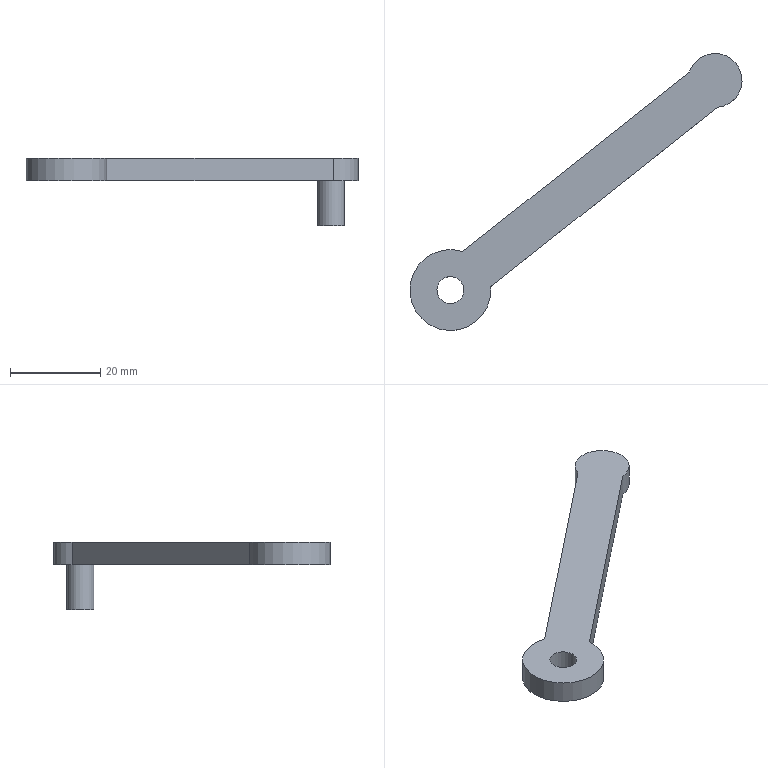Component | NX | CONN_ARM | 1 solid | 9 faces | box 73.78 x 61.58 x 15 mm | volume 5043 mm3 | plane 5 | cylinder 4 | commonest cylinder face diameters 6 x2 12 x1 18 x1
STEP:
#1=CARTESIAN_POINT('',(0.,0.,0.));
#2=DIRECTION('',(0.,0.,1.));
#3=DIRECTION('',(1.,0.,0.));
#4=AXIS2_PLACEMENT_3D('',#1,#2,#3);
#5=CARTESIAN_POINT('',(-109.814,-45.848,12.5));
#6=VERTEX_POINT('',#5);
#7=CARTESIAN_POINT('',(-59.494,-5.979,12.5));
#8=VERTEX_POINT('',#7);
#9=CARTESIAN_POINT('',(-109.814,-45.848,12.5));
#10=DIRECTION('',(0.7838,0.621,0.));
#11=VECTOR('',#10,1.);
#12=LINE('',#9,#11);
#13=CARTESIAN_POINT('',(-109.814,-45.848,7.5));
#14=DIRECTION('',(0.621,-0.7838,0.));
#15=DIRECTION('',(0.,0.,-1.));
#16=AXIS2_PLACEMENT_3D('',#13,#14,#15);
#17=PLANE('',#16);
#18=CARTESIAN_POINT('',(-5.,0.));
#19=DIRECTION('',(0.,1.));
#20=VECTOR('',#19,1.);
#21=LINE('',#18,#20);
#22=(GEOMETRIC_REPRESENTATION_CONTEXT(2)PARAMETRIC_REPRESENTATION_CONTEXT()REPRESENTATION_CONTEXT('',''));
#23=DEFINITIONAL_REPRESENTATION('',(#21),#22);
#24=PCURVE('',#17,#23);
#25=CARTESIAN_POINT('',(-60.,-0.,12.5));
#26=DIRECTION('',(0.,0.,1.));
#27=DIRECTION('',(-0.7838,-0.621,0.));
#28=AXIS2_PLACEMENT_3D('',#25,#26,#27);
#29=PLANE('',#28);
#30=CARTESIAN_POINT('',(67.517,5.));
#31=DIRECTION('',(-1.,0.));
#32=VECTOR('',#31,1.);
#33=LINE('',#30,#32);
#34=(GEOMETRIC_REPRESENTATION_CONTEXT(2)PARAMETRIC_REPRESENTATION_CONTEXT()REPRESENTATION_CONTEXT('',''));
#35=DEFINITIONAL_REPRESENTATION('',(#33),#34);
#36=PCURVE('',#29,#35);
#37=SURFACE_CURVE('',#12,(#24,#36),.PCURVE_S1.);
#38=EDGE_CURVE('',#6,#8,#37,.T.);
#39=ORIENTED_EDGE('',*,*,#38,.F.);
#40=CARTESIAN_POINT('',(-109.814,-45.848,7.5));
#41=VERTEX_POINT('',#40);
#42=CARTESIAN_POINT('',(-109.814,-45.848,7.5));
#43=DIRECTION('',(0.,0.,1.));
#44=VECTOR('',#43,1.);
#45=LINE('',#42,#44);
#46=CARTESIAN_POINT('',(0.,0.));
#47=DIRECTION('',(-1.,0.));
#48=VECTOR('',#47,1.);
#49=LINE('',#46,#48);
#50=(GEOMETRIC_REPRESENTATION_CONTEXT(2)PARAMETRIC_REPRESENTATION_CONTEXT()REPRESENTATION_CONTEXT('',''));
#51=DEFINITIONAL_REPRESENTATION('',(#49),#50);
#52=PCURVE('',#17,#51);
#53=CARTESIAN_POINT('',(-118.784,-46.577,7.5));
#54=DIRECTION('',(0.,0.,1.));
#55=DIRECTION('',(-0.7838,-0.621,0.));
#56=AXIS2_PLACEMENT_3D('',#53,#54,#55);
#57=CYLINDRICAL_SURFACE('',#56,9.);
#58=CARTESIAN_POINT('',(8.836,0.));
#59=DIRECTION('',(0.,1.));
#60=VECTOR('',#59,1.);
#61=LINE('',#58,#60);
#62=(GEOMETRIC_REPRESENTATION_CONTEXT(2)PARAMETRIC_REPRESENTATION_CONTEXT()REPRESENTATION_CONTEXT('',''));
#63=DEFINITIONAL_REPRESENTATION('',(#61),#62);
#64=PCURVE('',#57,#63);
#65=SURFACE_CURVE('',#45,(#52,#64),.PCURVE_S1.);
#66=EDGE_CURVE('',#41,#6,#65,.T.);
#67=ORIENTED_EDGE('',*,*,#66,.F.);
#68=CARTESIAN_POINT('',(-59.494,-5.979,7.5));
#69=VERTEX_POINT('',#68);
#70=CARTESIAN_POINT('',(-109.814,-45.848,7.5));
#71=DIRECTION('',(0.7838,0.621,0.));
#72=VECTOR('',#71,1.);
#73=LINE('',#70,#72);
#74=CARTESIAN_POINT('',(0.,0.));
#75=DIRECTION('',(0.,1.));
#76=VECTOR('',#75,1.);
#77=LINE('',#74,#76);
#78=(GEOMETRIC_REPRESENTATION_CONTEXT(2)PARAMETRIC_REPRESENTATION_CONTEXT()REPRESENTATION_CONTEXT('',''));
#79=DEFINITIONAL_REPRESENTATION('',(#77),#78);
#80=PCURVE('',#17,#79);
#81=CARTESIAN_POINT('',(-60.,-0.,7.5));
#82=DIRECTION('',(0.,0.,1.));
#83=DIRECTION('',(-0.7838,-0.621,0.));
#84=AXIS2_PLACEMENT_3D('',#81,#82,#83);
#85=PLANE('',#84);
#86=CARTESIAN_POINT('',(67.517,5.));
#87=DIRECTION('',(-1.,0.));
#88=VECTOR('',#87,1.);
#89=LINE('',#86,#88);
#90=(GEOMETRIC_REPRESENTATION_CONTEXT(2)PARAMETRIC_REPRESENTATION_CONTEXT()REPRESENTATION_CONTEXT('',''));
#91=DEFINITIONAL_REPRESENTATION('',(#89),#90);
#92=PCURVE('',#85,#91);
#93=SURFACE_CURVE('',#73,(#80,#92),.PCURVE_S1.);
#94=EDGE_CURVE('',#41,#69,#93,.T.);
#95=ORIENTED_EDGE('',*,*,#94,.T.);
#96=CARTESIAN_POINT('',(-59.494,-5.979,7.5));
#97=DIRECTION('',(0.,0.,1.));
#98=VECTOR('',#97,1.);
#99=LINE('',#96,#98);
#100=CARTESIAN_POINT('',(0.,64.2));
#101=DIRECTION('',(-1.,0.));
#102=VECTOR('',#101,1.);
#103=LINE('',#100,#102);
#104=(GEOMETRIC_REPRESENTATION_CONTEXT(2)PARAMETRIC_REPRESENTATION_CONTEXT()REPRESENTATION_CONTEXT('',''));
#105=DEFINITIONAL_REPRESENTATION('',(#103),#104);
#106=PCURVE('',#17,#105);
#107=CARTESIAN_POINT('',(-60.,-0.,7.5));
#108=DIRECTION('',(0.,0.,1.));
#109=DIRECTION('',(-0.7838,-0.621,0.));
#110=AXIS2_PLACEMENT_3D('',#107,#108,#109);
#111=CYLINDRICAL_SURFACE('',#110,6.);
#112=CARTESIAN_POINT('',(0.9851,0.));
#113=DIRECTION('',(0.,1.));
#114=VECTOR('',#113,1.);
#115=LINE('',#112,#114);
#116=(GEOMETRIC_REPRESENTATION_CONTEXT(2)PARAMETRIC_REPRESENTATION_CONTEXT()REPRESENTATION_CONTEXT('',''));
#117=DEFINITIONAL_REPRESENTATION('',(#115),#116);
#118=PCURVE('',#111,#117);
#119=SURFACE_CURVE('',#99,(#106,#118),.PCURVE_S1.);
#120=EDGE_CURVE('',#69,#8,#119,.T.);
#121=ORIENTED_EDGE('',*,*,#120,.T.);
#122=EDGE_LOOP('',(#39,#67,#95,#121));
#123=FACE_BOUND('',#122,.T.);
#124=ADVANCED_FACE('',(#123),#17,.T.);
#125=CARTESIAN_POINT('',(-65.705,1.859,12.5));
#126=VERTEX_POINT('',#125);
#127=CARTESIAN_POINT('',(-60.,-0.,12.5));
#128=DIRECTION('',(0.,0.,1.));
#129=DIRECTION('',(0.7838,0.621,0.));
#130=AXIS2_PLACEMENT_3D('',#127,#128,#129);
#131=CIRCLE('',#130,6.);
#132=CARTESIAN_POINT('',(-3.142,5.));
#133=DIRECTION('',(1.,0.));
#134=VECTOR('',#133,1.);
#135=LINE('',#132,#134);
#136=(GEOMETRIC_REPRESENTATION_CONTEXT(2)PARAMETRIC_REPRESENTATION_CONTEXT()REPRESENTATION_CONTEXT('',''));
#137=DEFINITIONAL_REPRESENTATION('',(#135),#136);
#138=PCURVE('',#111,#137);
#139=CARTESIAN_POINT('',(0.,0.));
#140=DIRECTION('',(-1.,0.));
#141=AXIS2_PLACEMENT_2D('',#139,#140);
#142=CIRCLE('',#141,6.);
#143=(GEOMETRIC_REPRESENTATION_CONTEXT(2)PARAMETRIC_REPRESENTATION_CONTEXT()REPRESENTATION_CONTEXT('',''));
#144=DEFINITIONAL_REPRESENTATION('',(#142),#143);
#145=PCURVE('',#29,#144);
#146=SURFACE_CURVE('',#131,(#138,#145),.PCURVE_S1.);
#147=EDGE_CURVE('',#8,#126,#146,.T.);
#148=ORIENTED_EDGE('',*,*,#147,.F.);
#149=ORIENTED_EDGE('',*,*,#120,.F.);
#150=CARTESIAN_POINT('',(-65.705,1.859,7.5));
#151=VERTEX_POINT('',#150);
#152=CARTESIAN_POINT('',(-60.,-0.,7.5));
#153=DIRECTION('',(0.,0.,1.));
#154=DIRECTION('',(0.7838,0.621,0.));
#155=AXIS2_PLACEMENT_3D('',#152,#153,#154);
#156=CIRCLE('',#155,6.);
#157=CARTESIAN_POINT('',(-3.142,0.));
#158=DIRECTION('',(1.,0.));
#159=VECTOR('',#158,1.);
#160=LINE('',#157,#159);
#161=(GEOMETRIC_REPRESENTATION_CONTEXT(2)PARAMETRIC_REPRESENTATION_CONTEXT()REPRESENTATION_CONTEXT('',''));
#162=DEFINITIONAL_REPRESENTATION('',(#160),#161);
#163=PCURVE('',#111,#162);
#164=CARTESIAN_POINT('',(0.,0.));
#165=DIRECTION('',(-1.,0.));
#166=AXIS2_PLACEMENT_2D('',#164,#165);
#167=CIRCLE('',#166,6.);
#168=(GEOMETRIC_REPRESENTATION_CONTEXT(2)PARAMETRIC_REPRESENTATION_CONTEXT()REPRESENTATION_CONTEXT('',''));
#169=DEFINITIONAL_REPRESENTATION('',(#167),#168);
#170=PCURVE('',#85,#169);
#171=SURFACE_CURVE('',#156,(#163,#170),.PCURVE_S1.);
#172=EDGE_CURVE('',#69,#151,#171,.T.);
#173=ORIENTED_EDGE('',*,*,#172,.T.);
#174=CARTESIAN_POINT('',(-65.705,1.859,7.5));
#175=DIRECTION('',(0.,0.,1.));
#176=VECTOR('',#175,1.);
#177=LINE('',#174,#176);
#178=CARTESIAN_POINT('',(5.298,0.));
#179=DIRECTION('',(0.,1.));
#180=VECTOR('',#179,1.);
#181=LINE('',#178,#180);
#182=(GEOMETRIC_REPRESENTATION_CONTEXT(2)PARAMETRIC_REPRESENTATION_CONTEXT()REPRESENTATION_CONTEXT('',''));
#183=DEFINITIONAL_REPRESENTATION('',(#181),#182);
#184=PCURVE('',#111,#183);
#185=CARTESIAN_POINT('',(-65.705,1.859,7.5));
#186=DIRECTION('',(-0.621,0.7838,0.));
#187=DIRECTION('',(0.,0.,1.));
#188=AXIS2_PLACEMENT_3D('',#185,#186,#187);
#189=PLANE('',#188);
#190=CARTESIAN_POINT('',(0.,0.));
#191=DIRECTION('',(1.,0.));
#192=VECTOR('',#191,1.);
#193=LINE('',#190,#192);
#194=(GEOMETRIC_REPRESENTATION_CONTEXT(2)PARAMETRIC_REPRESENTATION_CONTEXT()REPRESENTATION_CONTEXT('',''));
#195=DEFINITIONAL_REPRESENTATION('',(#193),#194);
#196=PCURVE('',#189,#195);
#197=SURFACE_CURVE('',#177,(#184,#196),.PCURVE_S1.);
#198=EDGE_CURVE('',#151,#126,#197,.T.);
#199=ORIENTED_EDGE('',*,*,#198,.T.);
#200=EDGE_LOOP('',(#148,#149,#173,#199));
#201=FACE_BOUND('',#200,.T.);
#202=ADVANCED_FACE('',(#201),#111,.T.);
#203=CARTESIAN_POINT('',(-116.024,-38.011,12.5));
#204=VERTEX_POINT('',#203);
#205=CARTESIAN_POINT('',(-65.705,1.859,12.5));
#206=DIRECTION('',(-0.7838,-0.621,0.));
#207=VECTOR('',#206,1.);
#208=LINE('',#205,#207);
#209=CARTESIAN_POINT('',(5.,0.));
#210=DIRECTION('',(0.,-1.));
#211=VECTOR('',#210,1.);
#212=LINE('',#209,#211);
#213=(GEOMETRIC_REPRESENTATION_CONTEXT(2)PARAMETRIC_REPRESENTATION_CONTEXT()REPRESENTATION_CONTEXT('',''));
#214=DEFINITIONAL_REPRESENTATION('',(#212),#213);
#215=PCURVE('',#189,#214);
#216=CARTESIAN_POINT('',(3.317,-5.));
#217=DIRECTION('',(1.,0.));
#218=VECTOR('',#217,1.);
#219=LINE('',#216,#218);
#220=(GEOMETRIC_REPRESENTATION_CONTEXT(2)PARAMETRIC_REPRESENTATION_CONTEXT()REPRESENTATION_CONTEXT('',''));
#221=DEFINITIONAL_REPRESENTATION('',(#219),#220);
#222=PCURVE('',#29,#221);
#223=SURFACE_CURVE('',#208,(#215,#222),.PCURVE_S1.);
#224=EDGE_CURVE('',#126,#204,#223,.T.);
#225=ORIENTED_EDGE('',*,*,#224,.F.);
#226=ORIENTED_EDGE('',*,*,#198,.F.);
#227=CARTESIAN_POINT('',(-116.024,-38.011,7.5));
#228=VERTEX_POINT('',#227);
#229=CARTESIAN_POINT('',(-65.705,1.859,7.5));
#230=DIRECTION('',(-0.7838,-0.621,0.));
#231=VECTOR('',#230,1.);
#232=LINE('',#229,#231);
#233=CARTESIAN_POINT('',(0.,0.));
#234=DIRECTION('',(0.,-1.));
#235=VECTOR('',#234,1.);
#236=LINE('',#233,#235);
#237=(GEOMETRIC_REPRESENTATION_CONTEXT(2)PARAMETRIC_REPRESENTATION_CONTEXT()REPRESENTATION_CONTEXT('',''));
#238=DEFINITIONAL_REPRESENTATION('',(#236),#237);
#239=PCURVE('',#189,#238);
#240=CARTESIAN_POINT('',(3.317,-5.));
#241=DIRECTION('',(1.,0.));
#242=VECTOR('',#241,1.);
#243=LINE('',#240,#242);
#244=(GEOMETRIC_REPRESENTATION_CONTEXT(2)PARAMETRIC_REPRESENTATION_CONTEXT()REPRESENTATION_CONTEXT('',''));
#245=DEFINITIONAL_REPRESENTATION('',(#243),#244);
#246=PCURVE('',#85,#245);
#247=SURFACE_CURVE('',#232,(#239,#246),.PCURVE_S1.);
#248=EDGE_CURVE('',#151,#228,#247,.T.);
#249=ORIENTED_EDGE('',*,*,#248,.T.);
#250=CARTESIAN_POINT('',(-116.024,-38.011,7.5));
#251=DIRECTION('',(0.,0.,1.));
#252=VECTOR('',#251,1.);
#253=LINE('',#250,#252);
#254=CARTESIAN_POINT('',(0.,-64.2));
#255=DIRECTION('',(1.,0.));
#256=VECTOR('',#255,1.);
#257=LINE('',#254,#256);
#258=(GEOMETRIC_REPRESENTATION_CONTEXT(2)PARAMETRIC_REPRESENTATION_CONTEXT()REPRESENTATION_CONTEXT('',''));
#259=DEFINITIONAL_REPRESENTATION('',(#257),#258);
#260=PCURVE('',#189,#259);
#261=CARTESIAN_POINT('',(3.731,0.));
#262=DIRECTION('',(0.,1.));
#263=VECTOR('',#262,1.);
#264=LINE('',#261,#263);
#265=(GEOMETRIC_REPRESENTATION_CONTEXT(2)PARAMETRIC_REPRESENTATION_CONTEXT()REPRESENTATION_CONTEXT('',''));
#266=DEFINITIONAL_REPRESENTATION('',(#264),#265);
#267=PCURVE('',#57,#266);
#268=SURFACE_CURVE('',#253,(#260,#267),.PCURVE_S1.);
#269=EDGE_CURVE('',#228,#204,#268,.T.);
#270=ORIENTED_EDGE('',*,*,#269,.T.);
#271=EDGE_LOOP('',(#225,#226,#249,#270));
#272=FACE_BOUND('',#271,.T.);
#273=ADVANCED_FACE('',(#272),#189,.T.);
#274=CARTESIAN_POINT('',(-118.784,-46.577,12.5));
#275=DIRECTION('',(0.,0.,1.));
#276=DIRECTION('',(0.7838,0.621,0.));
#277=AXIS2_PLACEMENT_3D('',#274,#275,#276);
#278=CIRCLE('',#277,9.);
#279=CARTESIAN_POINT('',(3.142,5.));
#280=DIRECTION('',(1.,0.));
#281=VECTOR('',#280,1.);
#282=LINE('',#279,#281);
#283=(GEOMETRIC_REPRESENTATION_CONTEXT(2)PARAMETRIC_REPRESENTATION_CONTEXT()REPRESENTATION_CONTEXT('',''));
#284=DEFINITIONAL_REPRESENTATION('',(#282),#283);
#285=PCURVE('',#57,#284);
#286=CARTESIAN_POINT('',(75.,0.));
#287=DIRECTION('',(-1.,0.));
#288=AXIS2_PLACEMENT_2D('',#286,#287);
#289=CIRCLE('',#288,9.);
#290=(GEOMETRIC_REPRESENTATION_CONTEXT(2)PARAMETRIC_REPRESENTATION_CONTEXT()REPRESENTATION_CONTEXT('',''));
#291=DEFINITIONAL_REPRESENTATION('',(#289),#290);
#292=PCURVE('',#29,#291);
#293=SURFACE_CURVE('',#278,(#285,#292),.PCURVE_S1.);
#294=EDGE_CURVE('',#204,#6,#293,.T.);
#295=ORIENTED_EDGE('',*,*,#294,.F.);
#296=ORIENTED_EDGE('',*,*,#269,.F.);
#297=CARTESIAN_POINT('',(-118.784,-46.577,7.5));
#298=DIRECTION('',(0.,0.,1.));
#299=DIRECTION('',(0.7838,0.621,0.));
#300=AXIS2_PLACEMENT_3D('',#297,#298,#299);
#301=CIRCLE('',#300,9.);
#302=CARTESIAN_POINT('',(3.142,0.));
#303=DIRECTION('',(1.,0.));
#304=VECTOR('',#303,1.);
#305=LINE('',#302,#304);
#306=(GEOMETRIC_REPRESENTATION_CONTEXT(2)PARAMETRIC_REPRESENTATION_CONTEXT()REPRESENTATION_CONTEXT('',''));
#307=DEFINITIONAL_REPRESENTATION('',(#305),#306);
#308=PCURVE('',#57,#307);
#309=CARTESIAN_POINT('',(75.,0.));
#310=DIRECTION('',(-1.,0.));
#311=AXIS2_PLACEMENT_2D('',#309,#310);
#312=CIRCLE('',#311,9.);
#313=(GEOMETRIC_REPRESENTATION_CONTEXT(2)PARAMETRIC_REPRESENTATION_CONTEXT()REPRESENTATION_CONTEXT('',''));
#314=DEFINITIONAL_REPRESENTATION('',(#312),#313);
#315=PCURVE('',#85,#314);
#316=SURFACE_CURVE('',#301,(#308,#315),.PCURVE_S1.);
#317=EDGE_CURVE('',#228,#41,#316,.T.);
#318=ORIENTED_EDGE('',*,*,#317,.T.);
#319=ORIENTED_EDGE('',*,*,#66,.T.);
#320=EDGE_LOOP('',(#295,#296,#318,#319));
#321=FACE_BOUND('',#320,.T.);
#322=ADVANCED_FACE('',(#321),#57,.T.);
#323=CARTESIAN_POINT('',(-116.433,-44.714,7.5));
#324=VERTEX_POINT('',#323);
#325=CARTESIAN_POINT('',(-118.784,-46.577,7.5));
#326=DIRECTION('',(0.,0.,1.));
#327=DIRECTION('',(0.7838,0.621,0.));
#328=AXIS2_PLACEMENT_3D('',#325,#326,#327);
#329=CIRCLE('',#328,3.);
#330=CARTESIAN_POINT('',(-118.784,-46.577,7.5));
#331=DIRECTION('',(0.,0.,1.));
#332=DIRECTION('',(-0.7838,-0.621,0.));
#333=AXIS2_PLACEMENT_3D('',#330,#331,#332);
#334=CYLINDRICAL_SURFACE('',#333,3.);
#335=CARTESIAN_POINT('',(3.142,0.));
#336=DIRECTION('',(1.,0.));
#337=VECTOR('',#336,1.);
#338=LINE('',#335,#337);
#339=(GEOMETRIC_REPRESENTATION_CONTEXT(2)PARAMETRIC_REPRESENTATION_CONTEXT()REPRESENTATION_CONTEXT('',''));
#340=DEFINITIONAL_REPRESENTATION('',(#338),#339);
#341=PCURVE('',#334,#340);
#342=CARTESIAN_POINT('',(75.,0.));
#343=DIRECTION('',(-1.,-0.));
#344=AXIS2_PLACEMENT_2D('',#342,#343);
#345=CIRCLE('',#344,3.);
#346=(GEOMETRIC_REPRESENTATION_CONTEXT(2)PARAMETRIC_REPRESENTATION_CONTEXT()REPRESENTATION_CONTEXT('',''));
#347=DEFINITIONAL_REPRESENTATION('',(#345),#346);
#348=PCURVE('',#85,#347);
#349=SURFACE_CURVE('',#329,(#341,#348),.PCURVE_S1.);
#350=EDGE_CURVE('',#324,#324,#349,.T.);
#351=ORIENTED_EDGE('',*,*,#350,.T.);
#352=CARTESIAN_POINT('',(-116.433,-44.714,12.5));
#353=VERTEX_POINT('',#352);
#354=CARTESIAN_POINT('',(-116.433,-44.714,7.5));
#355=CARTESIAN_POINT('',(-116.433,-44.714,12.5));
#356=B_SPLINE_CURVE_WITH_KNOTS('',1,(#354,#355),.UNSPECIFIED.,.F.,.F.,(2,2),(0.,5.),.PIECEWISE_BEZIER_KNOTS.);
#357=CARTESIAN_POINT('',(9.425,0.));
#358=DIRECTION('',(0.,1.));
#359=VECTOR('',#358,1.);
#360=LINE('',#357,#359);
#361=(GEOMETRIC_REPRESENTATION_CONTEXT(2)PARAMETRIC_REPRESENTATION_CONTEXT()REPRESENTATION_CONTEXT('',''));
#362=DEFINITIONAL_REPRESENTATION('',(#360),#361);
#363=PCURVE('',#334,#362);
#364=CARTESIAN_POINT('',(3.142,0.));
#365=DIRECTION('',(0.,1.));
#366=VECTOR('',#365,1.);
#367=LINE('',#364,#366);
#368=(GEOMETRIC_REPRESENTATION_CONTEXT(2)PARAMETRIC_REPRESENTATION_CONTEXT()REPRESENTATION_CONTEXT('',''));
#369=DEFINITIONAL_REPRESENTATION('',(#367),#368);
#370=PCURVE('',#334,#369);
#371=SEAM_CURVE('',#356,(#363,#370),.PCURVE_S1.);
#372=EDGE_CURVE('',#324,#353,#371,.T.);
#373=ORIENTED_EDGE('',*,*,#372,.T.);
#374=CARTESIAN_POINT('',(-118.784,-46.577,12.5));
#375=DIRECTION('',(0.,0.,1.));
#376=DIRECTION('',(0.7838,0.621,0.));
#377=AXIS2_PLACEMENT_3D('',#374,#375,#376);
#378=CIRCLE('',#377,3.);
#379=CARTESIAN_POINT('',(3.142,5.));
#380=DIRECTION('',(1.,0.));
#381=VECTOR('',#380,1.);
#382=LINE('',#379,#381);
#383=(GEOMETRIC_REPRESENTATION_CONTEXT(2)PARAMETRIC_REPRESENTATION_CONTEXT()REPRESENTATION_CONTEXT('',''));
#384=DEFINITIONAL_REPRESENTATION('',(#382),#383);
#385=PCURVE('',#334,#384);
#386=CARTESIAN_POINT('',(75.,0.));
#387=DIRECTION('',(-1.,-0.));
#388=AXIS2_PLACEMENT_2D('',#386,#387);
#389=CIRCLE('',#388,3.);
#390=(GEOMETRIC_REPRESENTATION_CONTEXT(2)PARAMETRIC_REPRESENTATION_CONTEXT()REPRESENTATION_CONTEXT('',''));
#391=DEFINITIONAL_REPRESENTATION('',(#389),#390);
#392=PCURVE('',#29,#391);
#393=SURFACE_CURVE('',#378,(#385,#392),.PCURVE_S1.);
#394=EDGE_CURVE('',#353,#353,#393,.T.);
#395=ORIENTED_EDGE('',*,*,#394,.F.);
#396=ORIENTED_EDGE('',*,*,#372,.F.);
#397=EDGE_LOOP('',(#351,#373,#395,#396));
#398=FACE_BOUND('',#397,.F.);
#399=ADVANCED_FACE('',(#398),#334,.F.);
#400=CARTESIAN_POINT('',(-57.649,1.863,7.5));
#401=VERTEX_POINT('',#400);
#402=CARTESIAN_POINT('',(-60.,-0.,7.5));
#403=DIRECTION('',(0.,0.,-1.));
#404=DIRECTION('',(0.7838,0.621,0.));
#405=AXIS2_PLACEMENT_3D('',#402,#403,#404);
#406=CIRCLE('',#405,3.);
#407=CARTESIAN_POINT('',(-3.,0.));
#408=CARTESIAN_POINT('',(-3.,5.196));
#409=CARTESIAN_POINT('',(1.5,2.598));
#410=CARTESIAN_POINT('',(6.,-0.));
#411=CARTESIAN_POINT('',(1.5,-2.598));
#412=CARTESIAN_POINT('',(-3.,-5.196));
#413=CARTESIAN_POINT('',(-3.,0.));
#414=(BOUNDED_CURVE()B_SPLINE_CURVE(2,(#407,#408,#409,#410,#411,#412,#413),.UNSPECIFIED.,.T.,.F.)B_SPLINE_CURVE_WITH_KNOTS((1,2,2,2,2,1),(-2.094,0.,2.094,4.189,6.283,8.378),.UNSPECIFIED.)CURVE()GEOMETRIC_REPRESENTATION_ITEM()RATIONAL_B_SPLINE_CURVE((1.,0.5,1.,0.5,1.,0.5,1.))REPRESENTATION_ITEM(''));
#415=(GEOMETRIC_REPRESENTATION_CONTEXT(2)PARAMETRIC_REPRESENTATION_CONTEXT()REPRESENTATION_CONTEXT('',''));
#416=DEFINITIONAL_REPRESENTATION('',(#414),#415);
#417=PCURVE('',#85,#416);
#418=CARTESIAN_POINT('',(-60.,-0.,-2.5));
#419=DIRECTION('',(0.,0.,1.));
#420=DIRECTION('',(-0.7838,-0.621,0.));
#421=AXIS2_PLACEMENT_3D('',#418,#419,#420);
#422=CYLINDRICAL_SURFACE('',#421,3.);
#423=CARTESIAN_POINT('',(9.425,10.));
#424=DIRECTION('',(-1.,0.));
#425=VECTOR('',#424,1.);
#426=LINE('',#423,#425);
#427=(GEOMETRIC_REPRESENTATION_CONTEXT(2)PARAMETRIC_REPRESENTATION_CONTEXT()REPRESENTATION_CONTEXT('',''));
#428=DEFINITIONAL_REPRESENTATION('',(#426),#427);
#429=PCURVE('',#422,#428);
#430=SURFACE_CURVE('',#406,(#417,#429),.PCURVE_S1.);
#431=EDGE_CURVE('',#401,#401,#430,.T.);
#432=ORIENTED_EDGE('',*,*,#431,.F.);
#433=EDGE_LOOP('',(#432));
#434=FACE_BOUND('',#433,.T.);
#435=ORIENTED_EDGE('',*,*,#94,.F.);
#436=ORIENTED_EDGE('',*,*,#317,.F.);
#437=ORIENTED_EDGE('',*,*,#248,.F.);
#438=ORIENTED_EDGE('',*,*,#172,.F.);
#439=EDGE_LOOP('',(#435,#436,#437,#438));
#440=FACE_BOUND('',#439,.T.);
#441=ORIENTED_EDGE('',*,*,#350,.T.);
#442=EDGE_LOOP('',(#441));
#443=FACE_BOUND('',#442,.T.);
#444=ADVANCED_FACE('',(#434,#440,#443),#85,.F.);
#445=ORIENTED_EDGE('',*,*,#38,.T.);
#446=ORIENTED_EDGE('',*,*,#147,.T.);
#447=ORIENTED_EDGE('',*,*,#224,.T.);
#448=ORIENTED_EDGE('',*,*,#294,.T.);
#449=EDGE_LOOP('',(#445,#446,#447,#448));
#450=FACE_BOUND('',#449,.T.);
#451=ORIENTED_EDGE('',*,*,#394,.F.);
#452=EDGE_LOOP('',(#451));
#453=FACE_BOUND('',#452,.T.);
#454=ADVANCED_FACE('',(#450,#453),#29,.T.);
#455=CARTESIAN_POINT('',(-57.649,1.863,-2.5));
#456=VERTEX_POINT('',#455);
#457=CARTESIAN_POINT('',(-60.,-0.,-2.5));
#458=DIRECTION('',(0.,0.,-1.));
#459=DIRECTION('',(0.7838,0.621,0.));
#460=AXIS2_PLACEMENT_3D('',#457,#458,#459);
#461=CIRCLE('',#460,3.);
#462=CARTESIAN_POINT('',(9.425,0.));
#463=DIRECTION('',(-1.,0.));
#464=VECTOR('',#463,1.);
#465=LINE('',#462,#464);
#466=(GEOMETRIC_REPRESENTATION_CONTEXT(2)PARAMETRIC_REPRESENTATION_CONTEXT()REPRESENTATION_CONTEXT('',''));
#467=DEFINITIONAL_REPRESENTATION('',(#465),#466);
#468=PCURVE('',#422,#467);
#469=CARTESIAN_POINT('',(-60.,-0.,-2.5));
#470=DIRECTION('',(0.,0.,-1.));
#471=DIRECTION('',(0.7838,0.621,0.));
#472=AXIS2_PLACEMENT_3D('',#469,#470,#471);
#473=PLANE('',#472);
#474=CARTESIAN_POINT('',(0.,0.));
#475=DIRECTION('',(1.,0.));
#476=AXIS2_PLACEMENT_2D('',#474,#475);
#477=CIRCLE('',#476,3.);
#478=(GEOMETRIC_REPRESENTATION_CONTEXT(2)PARAMETRIC_REPRESENTATION_CONTEXT()REPRESENTATION_CONTEXT('',''));
#479=DEFINITIONAL_REPRESENTATION('',(#477),#478);
#480=PCURVE('',#473,#479);
#481=SURFACE_CURVE('',#461,(#468,#480),.PCURVE_S1.);
#482=EDGE_CURVE('',#456,#456,#481,.T.);
#483=ORIENTED_EDGE('',*,*,#482,.F.);
#484=CARTESIAN_POINT('',(-57.649,1.863,-2.5));
#485=CARTESIAN_POINT('',(-57.649,1.863,7.5));
#486=B_SPLINE_CURVE_WITH_KNOTS('',1,(#484,#485),.UNSPECIFIED.,.F.,.F.,(2,2),(0.,10.),.PIECEWISE_BEZIER_KNOTS.);
#487=CARTESIAN_POINT('',(9.425,0.));
#488=DIRECTION('',(0.,1.));
#489=VECTOR('',#488,1.);
#490=LINE('',#487,#489);
#491=(GEOMETRIC_REPRESENTATION_CONTEXT(2)PARAMETRIC_REPRESENTATION_CONTEXT()REPRESENTATION_CONTEXT('',''));
#492=DEFINITIONAL_REPRESENTATION('',(#490),#491);
#493=PCURVE('',#422,#492);
#494=CARTESIAN_POINT('',(3.142,0.));
#495=DIRECTION('',(0.,1.));
#496=VECTOR('',#495,1.);
#497=LINE('',#494,#496);
#498=(GEOMETRIC_REPRESENTATION_CONTEXT(2)PARAMETRIC_REPRESENTATION_CONTEXT()REPRESENTATION_CONTEXT('',''));
#499=DEFINITIONAL_REPRESENTATION('',(#497),#498);
#500=PCURVE('',#422,#499);
#501=SEAM_CURVE('',#486,(#493,#500),.PCURVE_S1.);
#502=EDGE_CURVE('',#456,#401,#501,.T.);
#503=ORIENTED_EDGE('',*,*,#502,.T.);
#504=ORIENTED_EDGE('',*,*,#431,.T.);
#505=ORIENTED_EDGE('',*,*,#502,.F.);
#506=EDGE_LOOP('',(#483,#503,#504,#505));
#507=FACE_BOUND('',#506,.T.);
#508=ADVANCED_FACE('',(#507),#422,.T.);
#509=ORIENTED_EDGE('',*,*,#482,.T.);
#510=EDGE_LOOP('',(#509));
#511=FACE_BOUND('',#510,.T.);
#512=ADVANCED_FACE('',(#511),#473,.T.);
#513=CLOSED_SHELL('',(#124,#202,#273,#322,#399,#444,#454,#508,#512));
#514=MANIFOLD_SOLID_BREP('',#513);
#515=(LENGTH_UNIT()NAMED_UNIT(*)SI_UNIT(.MILLI.,.METRE.));
#516=UNCERTAINTY_MEASURE_WITH_UNIT(LENGTH_MEASURE(0.000002),#515,'','');
#517=(NAMED_UNIT(*)PLANE_ANGLE_UNIT()SI_UNIT($,.RADIAN.));
#518=(NAMED_UNIT(*)SI_UNIT($,.STERADIAN.)SOLID_ANGLE_UNIT());
#519=(GEOMETRIC_REPRESENTATION_CONTEXT(3)GLOBAL_UNCERTAINTY_ASSIGNED_CONTEXT((#516))GLOBAL_UNIT_ASSIGNED_CONTEXT((#515,#517,#518))REPRESENTATION_CONTEXT('',''));
#520=ADVANCED_BREP_SHAPE_REPRESENTATION('',(#4,#514),#519);